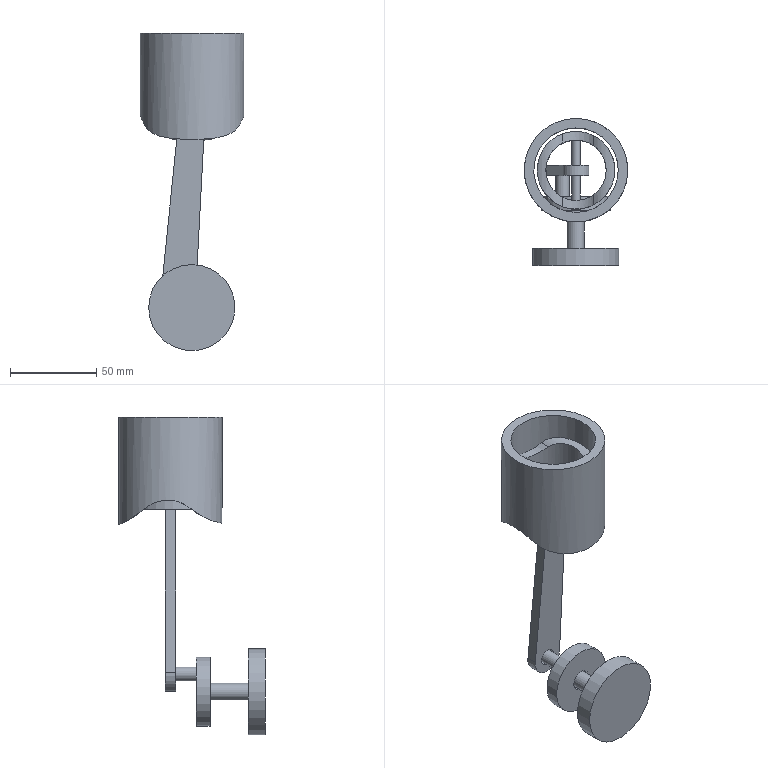Assembly | NX | mm | 6 component files | 6 solids | 38 faces | box 60 x 85 x 184.13 mm | volume 120144 mm3 | cylinder 24 | plane 14 | commonest cylinder face diameters 5 x3 10 x2 40.874 x2 27.799 x2 20 x1 15 x1 6 x1 50 x1
Bill of materials:
unnamed part 1 | 1 |  | Thin-walled open cylindrical tube with a flat top end. The other end has a curved saddle-shaped notch cut into it.
unnamed part 2 | 1 |  | Flat, slightly tapered link or bar of even thickness. Both ends are rounded and each has a through-hole; one hole is larger than the other.
unnamed part 3 | 1 |  | Plain solid cylindrical rod with flat ends.
unnamed part 4 | 1 |  | Flanged part: a thick circular disc with a central through-hole and a smaller cylindrical boss sticking out from one face.
unnamed part 5 | 1 |  | Solid disc head with a smaller solid cylindrical shank in the middle of one face, forming a T-shaped profile like a knob or headed pin.
unnamed part 6 | 1 |  | Short thin-walled cylindrical sleeve with a saddle-shaped notched top end, a flat bottom end, and one small radial hole through the wall near the bottom.
Mates:
1. fix | base_plate 1 component
2. touch align | crank 1 face | base_plate 1 face
3. touch align | crank 1 face | base_plate 1 face
4. touch align | connecting_rod 1 face | crank 1 face
5. touch align | connecting_rod 1 face | crank 1 face
6. touch align | pin 1 face | connecting_rod 1 face
7. center | pin 1 face | pin 1 face | connecting_rod 1 face | connecting_rod 1 face
8. touch align | piston 1 face | pin 1 face
9. touch align | piston 1 face | pin 1 face
10. touch align | cylinder 1 face | piston 1 face
11. fix | cylinder 1 component